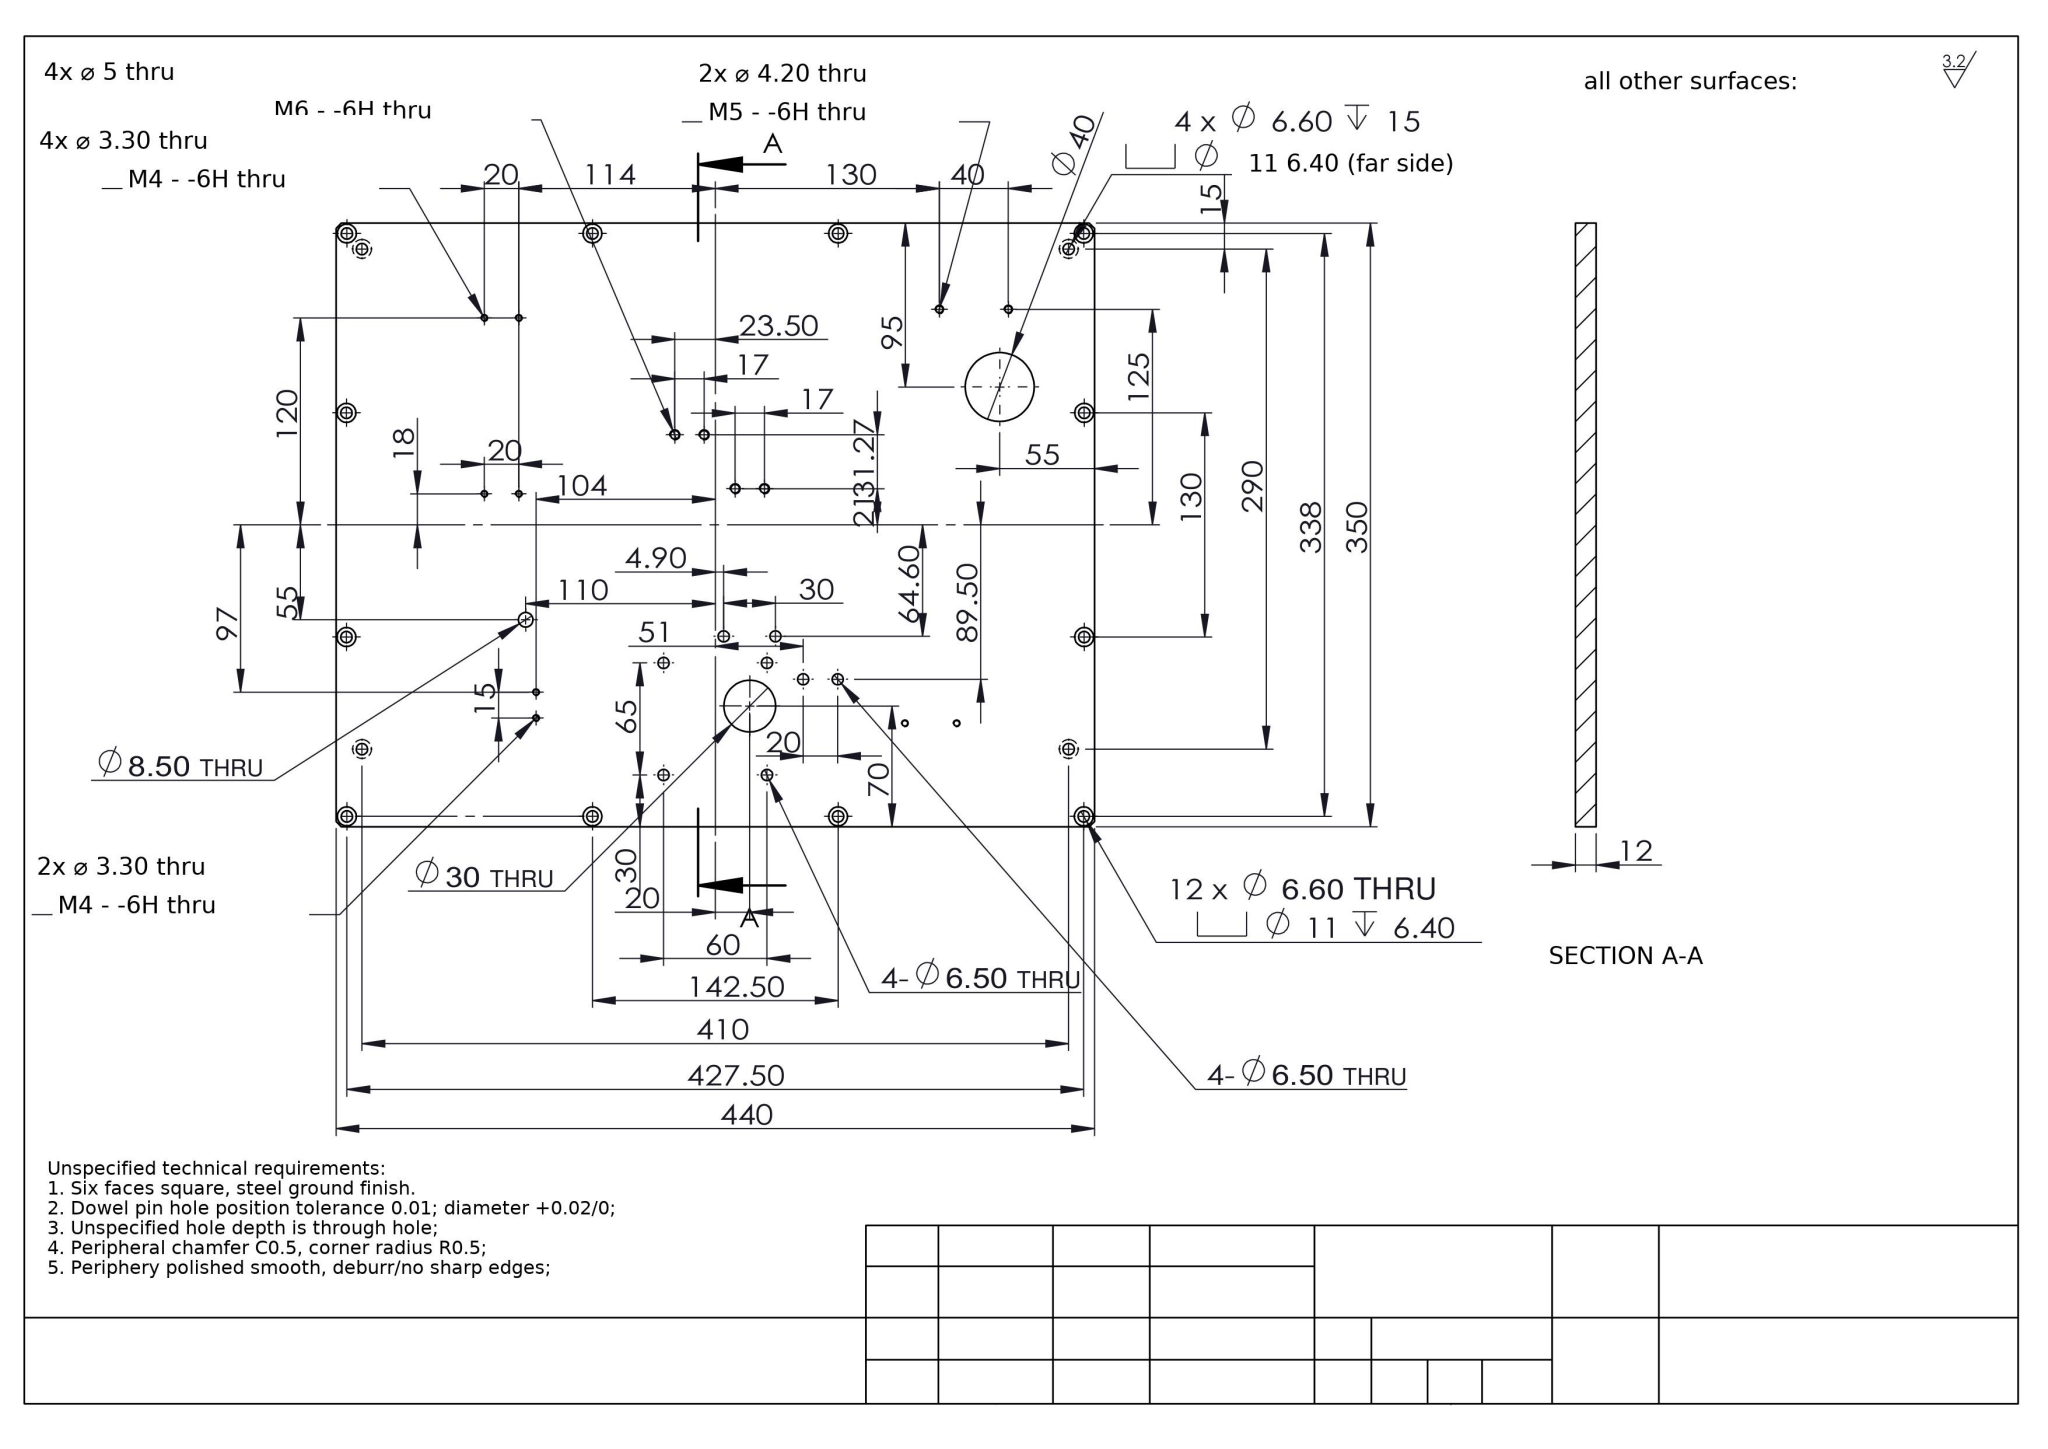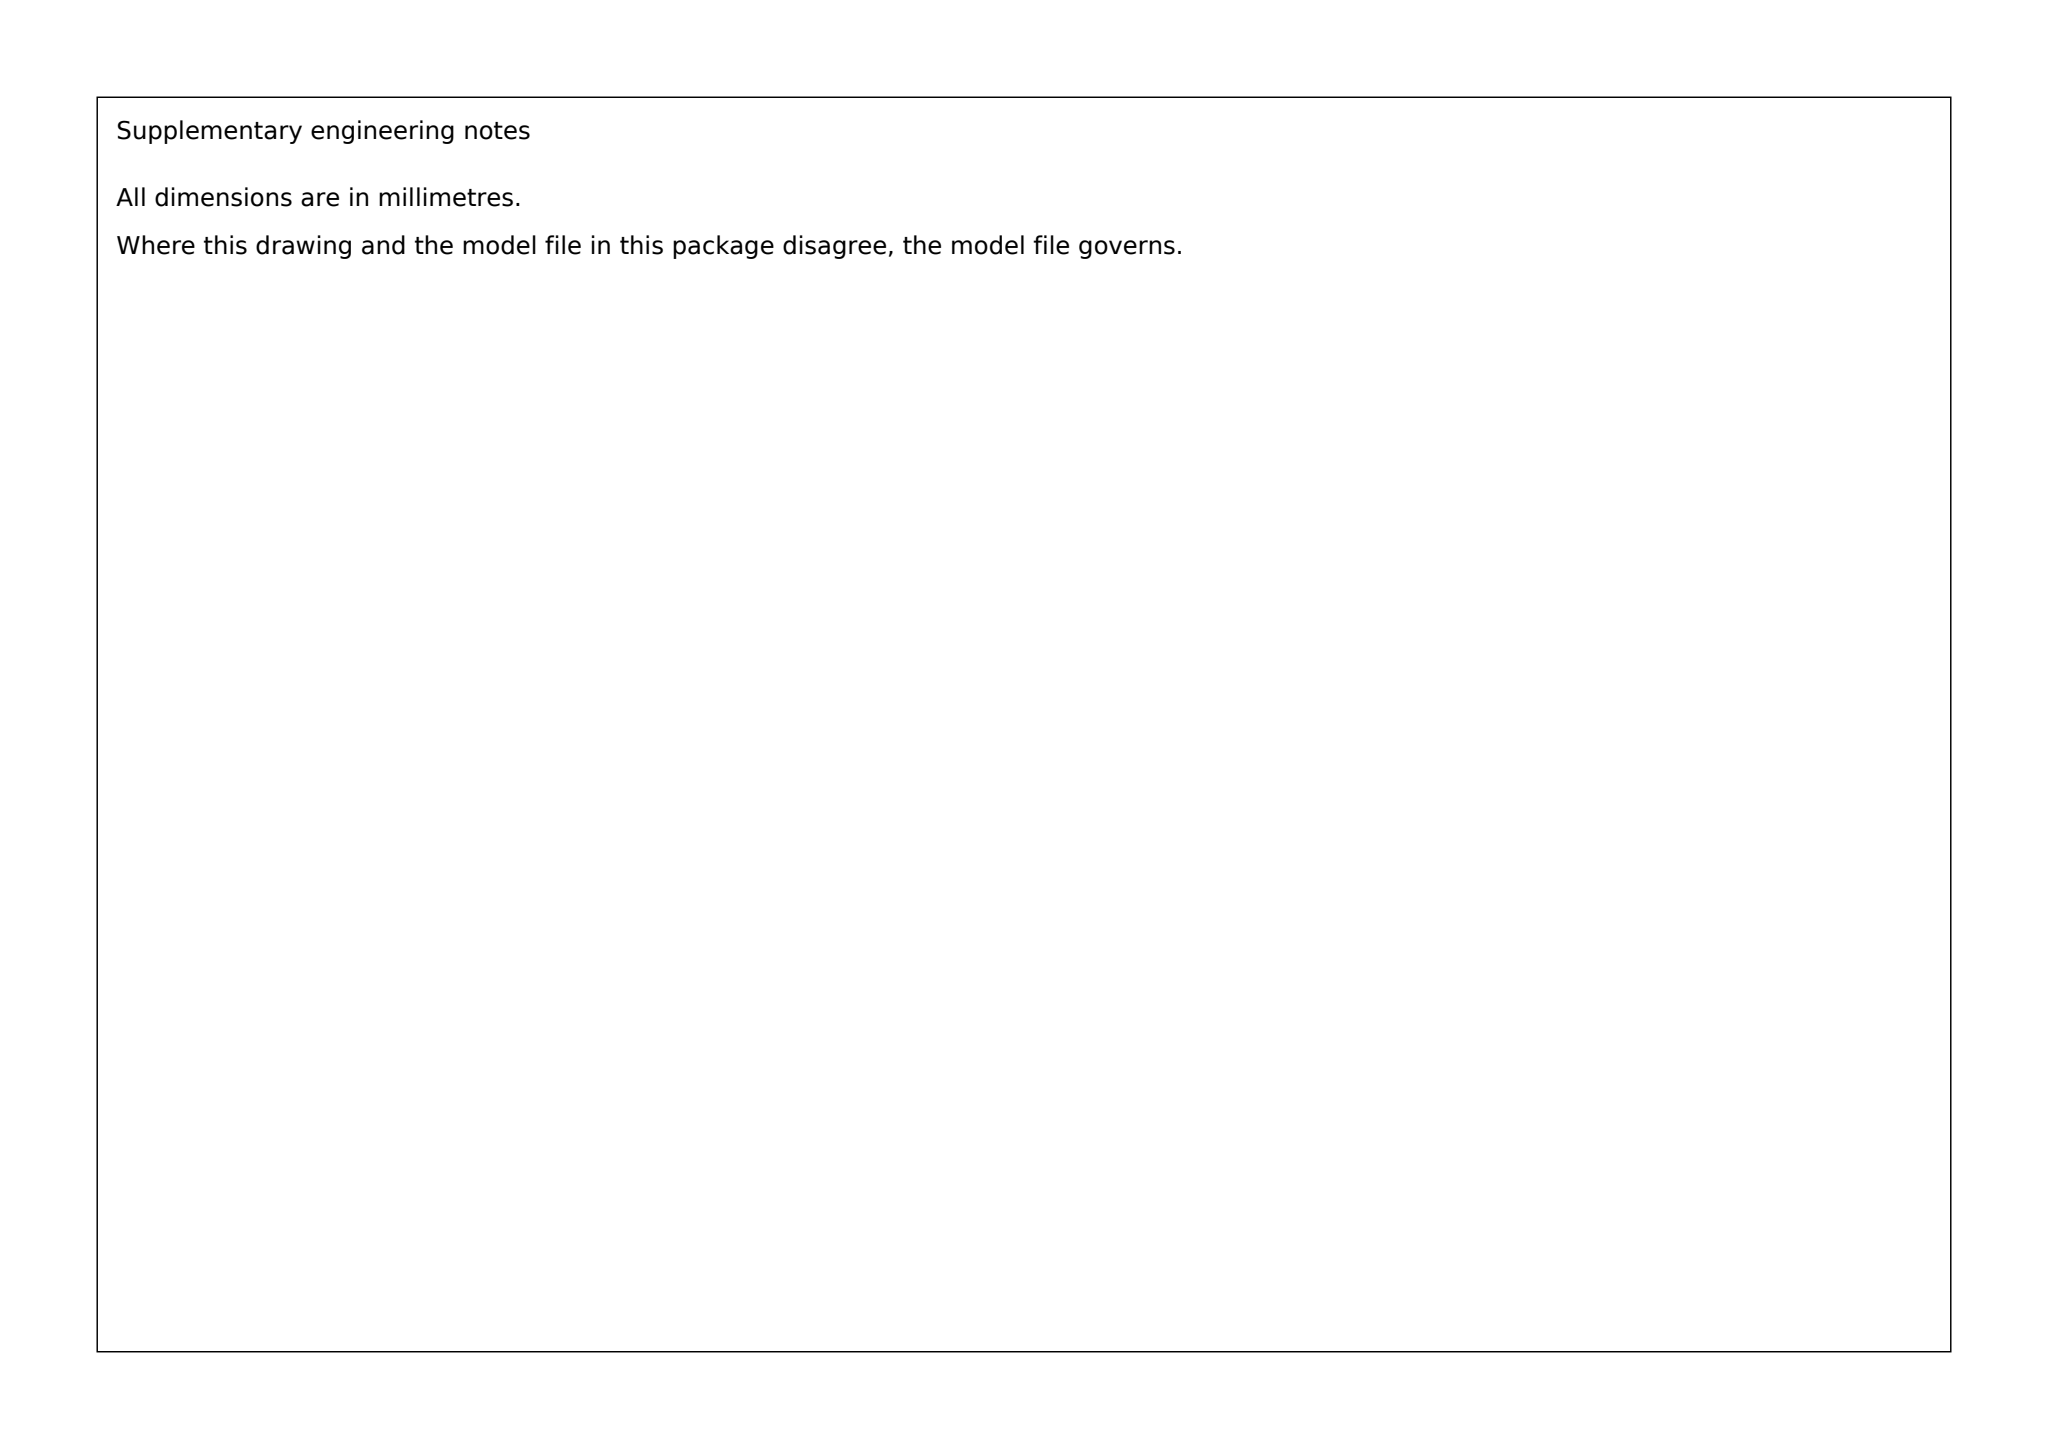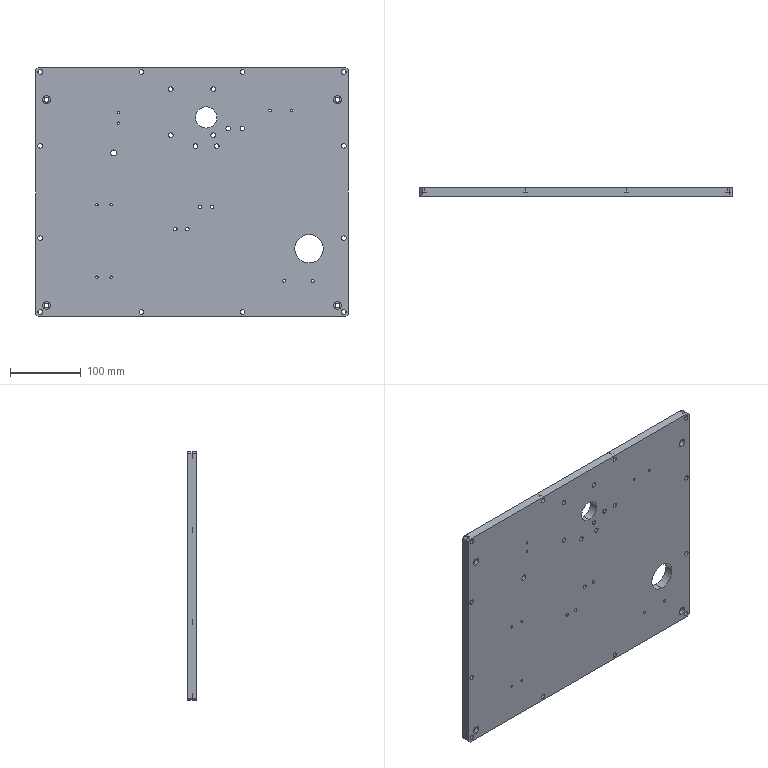Part | SolidWorks | mm | 1 solid | 140 faces | box 440 x 12 x 350 mm | volume 1805463 mm3 | cylinder 114 | plane 26 | commonest cylinder face diameters 11 x32 6.6 x32 3.3 x16 6.5 x16 5 x8 4.2 x4 40 x2 8.5 x2
build123d program:
from build123d import *

# Parameters (mm, degrees)
SKETCH1_W                                       = 440
SKETCH1_H                                       = 350
BOSS_EXTRUDE1_DEPTH                             = 12
SKETCH7_R                                       = 15
CUT_EXTRUDE2_DEPTH                              = 282.37
SKETCH8_R                                       = 4.25
CUT_EXTRUDE3_DEPTH                              = 282.37
SKETCH9_R                                       = 3.25
CUT_EXTRUDE4_DEPTH                              = 282.37
M4_TAPPED_HOLE3_D                               = 3.3
SKETCH12_R                                      = 3.25
CUT_EXTRUDE5_DEPTH                              = 282.37
M6_HEX_SOCKET_HEAD_CAP_SCREW_CBORE1_D           = 6.6
M6_HEX_SOCKET_HEAD_CAP_SCREW_CBORE1_CBORE_D     = 11
M6_HEX_SOCKET_HEAD_CAP_SCREW_CBORE1_CBORE_DEPTH = 6.4
M6_HEX_SOCKET_HEAD_CAP_SCREW_CBORE2_D           = 6.6
M6_HEX_SOCKET_HEAD_CAP_SCREW_CBORE2_CBORE_D     = 11
M6_HEX_SOCKET_HEAD_CAP_SCREW_CBORE2_CBORE_DEPTH = 6.4
LPATTERN3_COUNT                                 = 2
LPATTERN3_PITCH                                 = 142.5
MIRROR6_COPY_1_D                                = 6.6
MIRROR6_COPY_1_CBORE_D                          = 11
MIRROR6_COPY_1_CBORE_DEPTH                      = 6.4
MIRROR7_COPY_1_D                                = 6.6
MIRROR7_COPY_1_CBORE_D                          = 11
MIRROR7_COPY_1_CBORE_DEPTH                      = 6.4
MIRROR7_COPY_2_D                                = 6.6
MIRROR7_COPY_2_CBORE_D                          = 11
MIRROR7_COPY_2_CBORE_DEPTH                      = 6.4
MIRROR7_COPY_3_D                                = 6.6
MIRROR7_COPY_3_CBORE_D                          = 11
MIRROR7_COPY_3_CBORE_DEPTH                      = 6.4
MIRROR8_COPY_1_D                                = 6.6
MIRROR8_COPY_1_CBORE_D                          = 11
MIRROR8_COPY_1_CBORE_DEPTH                      = 6.4
CHAMFER1_SIZE                                   = 3
M5_TAPPED_HOLE1_D                               = 4.2
M4_TAPPED_HOLE4_D                               = 3.3
M6_TAPPED_HOLE1_D                               = 5
SKETCH24_R                                      = 3.25
CUT_EXTRUDE6_DEPTH                              = 282.37
SKETCH25_R                                      = 3.25
CUT_EXTRUDE7_DEPTH                              = 282.37
M6_HEX_SOCKET_HEAD_CAP_SCREW_CBORE3_D           = 6.6
M6_HEX_SOCKET_HEAD_CAP_SCREW_CBORE3_DEPTH       = 15
M6_HEX_SOCKET_HEAD_CAP_SCREW_CBORE3_CBORE_D     = 11
M6_HEX_SOCKET_HEAD_CAP_SCREW_CBORE3_CBORE_DEPTH = 6.4
M6_HEX_SOCKET_HEAD_CAP_SCREW_CBORE3_TIP         = 1.983
SKETCH29_R                                      = 20
CUT_EXTRUDE9_DEPTH                              = 282.37
M4_TAPPED_HOLE5_D                               = 3.3


with BuildPart() as part:
    # Sketch1 → Boss-Extrude1 (new body)
    with BuildSketch(Plane(origin=(0, 0, 0), x_dir=(1, 0, 0), z_dir=(0, 1, 0))):
        Rectangle(SKETCH1_W, SKETCH1_H)
    extrude(amount=BOSS_EXTRUDE1_DEPTH)

    # Sketch7 → Cut-Extrude2 (cut, through all)
    with BuildSketch(Plane(origin=(0, 12, 0), x_dir=(1, 0, 0), z_dir=(0, 1, 0))):
        with Locations(Location((20, -105, 0), (0, 0, 270))):
            Circle(SKETCH7_R)
    extrude(amount=-CUT_EXTRUDE2_DEPTH, mode=Mode.SUBTRACT)

    # Sketch8 → Cut-Extrude3 (cut, through all)
    with BuildSketch(Plane(origin=(0, 12, 0), x_dir=(1, 0, 0), z_dir=(0, 1, 0))):
        with Locations(Location((-110, -55, 0), (0, 0, 270))):
            Circle(SKETCH8_R)
    extrude(amount=-CUT_EXTRUDE3_DEPTH, mode=Mode.SUBTRACT)

    # Sketch9 → Cut-Extrude4 (cut, through all)
    with BuildSketch(Plane.XZ):
        with Locations(Location((-30, 80, 0), (0, 0, 270))):
            Circle(SKETCH9_R)
        with Locations(Location((-30, 145, 0), (0, 0, 270))):
            Circle(SKETCH9_R)
        with Locations(Location((30, 145, 0), (0, 0, 270))):
            Circle(SKETCH9_R)
        with Locations(Location((30, 80, 0), (0, 0, 270))):
            Circle(SKETCH9_R)
    extrude(amount=-CUT_EXTRUDE4_DEPTH, mode=Mode.SUBTRACT)

    # M4 Tapped Hole3 (through all)
    with Locations(Plane(origin=(0, 12, 0), x_dir=(1, 0, 0), z_dir=(0, 1, 0))):
        with Locations((-104, -96.999), (-104, -111.999)):
            Hole(M4_TAPPED_HOLE3_D / 2)

    # Sketch12 → Cut-Extrude5 (cut, through all)
    with BuildSketch(Plane.XZ):
        with Locations(Location((51, 89.5, 0), (0, 0, 270))):
            Circle(SKETCH12_R)
        with Locations(Location((71, 89.5, 0), (0, 0, 270))):
            Circle(SKETCH12_R)
    extrude(amount=-CUT_EXTRUDE5_DEPTH, mode=Mode.SUBTRACT)

    # M6 Hex Socket Head Cap Screw CBORE1 (through all)
    with Locations(Plane(origin=(0, 12, 0), x_dir=(1, 0, 0), z_dir=(0, 1, 0))):
        with Locations((-71.25, -169)):
            m6_hex_socket_head_cap_screw_cbore1 = CounterBoreHole(M6_HEX_SOCKET_HEAD_CAP_SCREW_CBORE1_D / 2, M6_HEX_SOCKET_HEAD_CAP_SCREW_CBORE1_CBORE_D / 2, M6_HEX_SOCKET_HEAD_CAP_SCREW_CBORE1_CBORE_DEPTH)

    # M6 Hex Socket Head Cap Screw CBORE2 (through all)
    with Locations(Plane(origin=(0, 12, 0), x_dir=(1, 0, 0), z_dir=(0, 1, 0))):
        with Locations((-214, 65)):
            m6_hex_socket_head_cap_screw_cbore2 = CounterBoreHole(M6_HEX_SOCKET_HEAD_CAP_SCREW_CBORE2_D / 2, M6_HEX_SOCKET_HEAD_CAP_SCREW_CBORE2_CBORE_D / 2, M6_HEX_SOCKET_HEAD_CAP_SCREW_CBORE2_CBORE_DEPTH)

    # Mirror5: M6 Hex Socket Head Cap Screw CBORE2 across plane
    add(m6_hex_socket_head_cap_screw_cbore2.mirror(Plane.XY), mode=Mode.SUBTRACT)

    # LPattern3: M6 Hex Socket Head Cap Screw CBORE1 ×2
    with Locations(*[(-i * LPATTERN3_PITCH, 0, 0) for i in range(1, LPATTERN3_COUNT)]):
        add(m6_hex_socket_head_cap_screw_cbore1, mode=Mode.SUBTRACT)

    # Mirror6: M6 Hex Socket Head Cap Screw CBORE1 across plane
    add(m6_hex_socket_head_cap_screw_cbore1.mirror(Plane(origin=(0, 0, 0), x_dir=(0, 0, 1), z_dir=(1, 0, 0))), mode=Mode.SUBTRACT)

    # Mirror6 copy 1 (through all)
    with Locations(Plane(origin=(142.5, 12, 0), x_dir=(-1, 0, 0), z_dir=(0, 1, 0))):
        with Locations((-71.25, 169)):
            CounterBoreHole(MIRROR6_COPY_1_D / 2, MIRROR6_COPY_1_CBORE_D / 2, MIRROR6_COPY_1_CBORE_DEPTH)

    # Mirror7: M6 Hex Socket Head Cap Screw CBORE1 across plane
    add(m6_hex_socket_head_cap_screw_cbore1.mirror(Plane.XY), mode=Mode.SUBTRACT)

    # Mirror7 copy 1 (through all)
    with Locations(Plane(origin=(-142.5, 12, 0), x_dir=(1, 0, 0), z_dir=(0, 1, 0))):
        with Locations((-71.25, 169)):
            CounterBoreHole(MIRROR7_COPY_1_D / 2, MIRROR7_COPY_1_CBORE_D / 2, MIRROR7_COPY_1_CBORE_DEPTH)

    # Mirror7 copy 2 (through all)
    with Locations(Plane(origin=(0, 12, 0), x_dir=(-1, 0, 0), z_dir=(0, 1, 0))):
        with Locations((-71.25, -169)):
            CounterBoreHole(MIRROR7_COPY_2_D / 2, MIRROR7_COPY_2_CBORE_D / 2, MIRROR7_COPY_2_CBORE_DEPTH)

    # Mirror7 copy 3 (through all)
    with Locations(Plane(origin=(142.5, 12, 0), x_dir=(-1, 0, 0), z_dir=(0, 1, 0))):
        with Locations((-71.25, -169)):
            CounterBoreHole(MIRROR7_COPY_3_D / 2, MIRROR7_COPY_3_CBORE_D / 2, MIRROR7_COPY_3_CBORE_DEPTH)

    # Mirror8: M6 Hex Socket Head Cap Screw CBORE2 across plane
    add(m6_hex_socket_head_cap_screw_cbore2.mirror(Plane(origin=(0, 0, 0), x_dir=(0, 0, 1), z_dir=(1, 0, 0))), mode=Mode.SUBTRACT)

    # Mirror8 copy 1 (through all)
    with Locations(Plane(origin=(0, 12, 0), x_dir=(-1, 0, 0), z_dir=(0, 1, 0))):
        with Locations((-214, 65)):
            CounterBoreHole(MIRROR8_COPY_1_D / 2, MIRROR8_COPY_1_CBORE_D / 2, MIRROR8_COPY_1_CBORE_DEPTH)

    # Chamfer1
    chamfer1_edges = [part.edges().sort_by_distance(p)[0] for p in [
        (220, 6, 175),
        (-220, 6, 175),
        (-220, 6, -175),
        (220, 6, -175),
    ]]
    chamfer(chamfer1_edges, length=CHAMFER1_SIZE)

    # M5 Tapped Hole1 (through all)
    with Locations(Plane(origin=(0, 12, 0), x_dir=(1, 0, 0), z_dir=(0, 1, 0))):
        with Locations((130, 125), (170, 125)):
            Hole(M5_TAPPED_HOLE1_D / 2)

    # M4 Tapped Hole4 (through all)
    with Locations(Plane(origin=(0, 12, 0), x_dir=(1, 0, 0), z_dir=(0, 1, 0))):
        with Locations((-134, 120), (-114, 120), (-134, 18), (-114, 18)):
            Hole(M4_TAPPED_HOLE4_D / 2)

    # M6 Tapped Hole1 (through all)
    with Locations(Plane(origin=(0, 12, 0), x_dir=(1, 0, 0), z_dir=(0, 1, 0))):
        with Locations((28.5, 21), (11.5, 21), (-23.5, 52.27), (-6.5, 52.27)):
            Hole(M6_TAPPED_HOLE1_D / 2)

    # Sketch24 → Cut-Extrude6 (cut, through all)
    with BuildSketch(Plane(origin=(0, 12, 0), x_dir=(1, 0, 0), z_dir=(0, 1, 0))):
        with Locations(Location((34.9, -64.6, 0), (0, 0, 270))):
            Circle(SKETCH24_R)
        with Locations(Location((4.9, -64.6, 0), (0, 0, 270))):
            Circle(SKETCH24_R)
    extrude(amount=-CUT_EXTRUDE6_DEPTH, mode=Mode.SUBTRACT)

    # Sketch25 → Cut-Extrude7 (cut, through all)
    with BuildSketch(Plane(origin=(0, 12, 0), x_dir=(1, 0, 0), z_dir=(0, 1, 0))):
        with Locations(Location((205, 160, 0), (0, 0, 270))):
            Circle(SKETCH25_R)
        with Locations(Location((205, -130, 0), (0, 0, 270))):
            Circle(SKETCH25_R)
        with Locations(Location((-205, 160, 0), (0, 0, 270))):
            Circle(SKETCH25_R)
        with Locations(Location((-205, -130, 0), (0, 0, 270))):
            Circle(SKETCH25_R)
    extrude(amount=-CUT_EXTRUDE7_DEPTH, mode=Mode.SUBTRACT)

    # M6 Hex Socket Head Cap Screw CBORE3
    with Locations(Plane(origin=(0, 0, 0), x_dir=(-1, 0, 0), z_dir=(0, -1, 0))):
        with Locations((-205, 160), (205, 160), (-205, -130), (205, -130)):
            CounterBoreHole(M6_HEX_SOCKET_HEAD_CAP_SCREW_CBORE3_D / 2, M6_HEX_SOCKET_HEAD_CAP_SCREW_CBORE3_CBORE_D / 2, M6_HEX_SOCKET_HEAD_CAP_SCREW_CBORE3_CBORE_DEPTH, depth=M6_HEX_SOCKET_HEAD_CAP_SCREW_CBORE3_DEPTH)
            with Locations((0, 0, -(M6_HEX_SOCKET_HEAD_CAP_SCREW_CBORE3_DEPTH + M6_HEX_SOCKET_HEAD_CAP_SCREW_CBORE3_TIP / 2))):  # 118° drill point
                Cone(0, M6_HEX_SOCKET_HEAD_CAP_SCREW_CBORE3_D / 2, M6_HEX_SOCKET_HEAD_CAP_SCREW_CBORE3_TIP, mode=Mode.SUBTRACT)

    # Sketch29 → Cut-Extrude9 (cut, through all)
    with BuildSketch(Plane(origin=(0, 12, 0), x_dir=(1, 0, 0), z_dir=(0, 1, 0))):
        with Locations(Location((165, 80, 0), (0, 0, 270))):
            Circle(SKETCH29_R)
    extrude(amount=-CUT_EXTRUDE9_DEPTH, mode=Mode.SUBTRACT)

    # M4 Tapped Hole5 (through all)
    with Locations(Plane(origin=(110, 12, 115), x_dir=(0, 0, 1), z_dir=(0, 1, 0))):
        with Locations((0, 0), (0, 30)):
            Hole(M4_TAPPED_HOLE5_D / 2)


solid = part.part